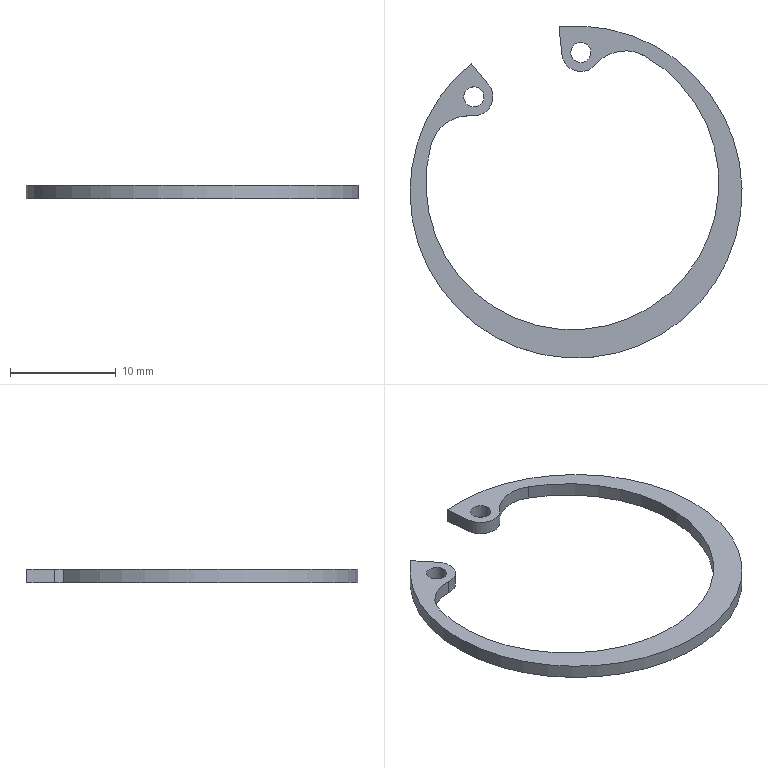Component | NX | 16 | 1 solid | 12 faces | box 31.4 x 31.4 x 1.3 mm | volume 239 mm3 | cylinder 8 | plane 4 | commonest cylinder face diameters 7.4 x2 3.6 x2 1.9 x2 27.7 x1 31.4 x1
STEP:
#1=CARTESIAN_POINT('',(0.,0.,0.));
#2=DIRECTION('',(0.,0.,1.));
#3=DIRECTION('',(1.,0.,0.));
#4=AXIS2_PLACEMENT_3D('',#1,#2,#3);
#5=CARTESIAN_POINT('',(-9.811,23.707,-49.8));
#6=VERTEX_POINT('',#5);
#7=CARTESIAN_POINT('',(-9.811,23.707,-48.5));
#8=VERTEX_POINT('',#7);
#9=CARTESIAN_POINT('',(-9.811,23.707,-49.8));
#10=DIRECTION('',(0.,0.,1.));
#11=VECTOR('',#10,1.);
#12=LINE('',#9,#11);
#13=CARTESIAN_POINT('',(-10.132,20.021,-49.8));
#14=DIRECTION('',(0.,0.,1.));
#15=DIRECTION('',(-0.9237,-0.383,0.));
#16=AXIS2_PLACEMENT_3D('',#13,#14,#15);
#17=CYLINDRICAL_SURFACE('',#16,3.7);
#18=CARTESIAN_POINT('',(4.233,0.));
#19=DIRECTION('',(0.,1.));
#20=VECTOR('',#19,1.);
#21=LINE('',#18,#20);
#22=(GEOMETRIC_REPRESENTATION_CONTEXT(2)PARAMETRIC_REPRESENTATION_CONTEXT()REPRESENTATION_CONTEXT('',''));
#23=DEFINITIONAL_REPRESENTATION('',(#21),#22);
#24=PCURVE('',#17,#23);
#25=CARTESIAN_POINT('',(-9.655,25.501,-49.8));
#26=DIRECTION('',(0.,0.,1.));
#27=DIRECTION('',(-0.9237,-0.383,0.));
#28=AXIS2_PLACEMENT_3D('',#25,#26,#27);
#29=CYLINDRICAL_SURFACE('',#28,1.8);
#30=CARTESIAN_POINT('',(1.091,0.));
#31=DIRECTION('',(0.,1.));
#32=VECTOR('',#31,1.);
#33=LINE('',#30,#32);
#34=(GEOMETRIC_REPRESENTATION_CONTEXT(2)PARAMETRIC_REPRESENTATION_CONTEXT()REPRESENTATION_CONTEXT('',''));
#35=DEFINITIONAL_REPRESENTATION('',(#33),#34);
#36=PCURVE('',#29,#35);
#37=SURFACE_CURVE('',#12,(#24,#36),.PCURVE_S1.);
#38=EDGE_CURVE('',#6,#8,#37,.T.);
#39=ORIENTED_EDGE('',*,*,#38,.F.);
#40=CARTESIAN_POINT('',(-13.699,21.002,-49.8));
#41=VERTEX_POINT('',#40);
#42=CARTESIAN_POINT('',(-10.132,20.021,-49.8));
#43=DIRECTION('',(0.,0.,1.));
#44=DIRECTION('',(0.9237,0.383,0.));
#45=AXIS2_PLACEMENT_3D('',#42,#43,#44);
#46=CIRCLE('',#45,3.7);
#47=CARTESIAN_POINT('',(3.142,0.));
#48=DIRECTION('',(1.,0.));
#49=VECTOR('',#48,1.);
#50=LINE('',#47,#49);
#51=(GEOMETRIC_REPRESENTATION_CONTEXT(2)PARAMETRIC_REPRESENTATION_CONTEXT()REPRESENTATION_CONTEXT('',''));
#52=DEFINITIONAL_REPRESENTATION('',(#50),#51);
#53=PCURVE('',#17,#52);
#54=CARTESIAN_POINT('',(-10.132,20.021,-49.8));
#55=DIRECTION('',(0.,0.,1.));
#56=DIRECTION('',(-0.9237,-0.383,0.));
#57=AXIS2_PLACEMENT_3D('',#54,#55,#56);
#58=PLANE('',#57);
#59=CARTESIAN_POINT('',(0.,0.));
#60=DIRECTION('',(-1.,0.));
#61=AXIS2_PLACEMENT_2D('',#59,#60);
#62=CIRCLE('',#61,3.7);
#63=(GEOMETRIC_REPRESENTATION_CONTEXT(2)PARAMETRIC_REPRESENTATION_CONTEXT()REPRESENTATION_CONTEXT('',''));
#64=DEFINITIONAL_REPRESENTATION('',(#62),#63);
#65=PCURVE('',#58,#64);
#66=SURFACE_CURVE('',#46,(#53,#65),.PCURVE_S1.);
#67=EDGE_CURVE('',#6,#41,#66,.T.);
#68=ORIENTED_EDGE('',*,*,#67,.T.);
#69=CARTESIAN_POINT('',(-13.699,21.002,-48.5));
#70=VERTEX_POINT('',#69);
#71=CARTESIAN_POINT('',(-13.699,21.002,-49.8));
#72=DIRECTION('',(0.,0.,1.));
#73=VECTOR('',#72,1.);
#74=LINE('',#71,#73);
#75=CARTESIAN_POINT('',(5.622,0.));
#76=DIRECTION('',(0.,1.));
#77=VECTOR('',#76,1.);
#78=LINE('',#75,#77);
#79=(GEOMETRIC_REPRESENTATION_CONTEXT(2)PARAMETRIC_REPRESENTATION_CONTEXT()REPRESENTATION_CONTEXT('',''));
#80=DEFINITIONAL_REPRESENTATION('',(#78),#79);
#81=PCURVE('',#17,#80);
#82=CARTESIAN_POINT('',(-0.3447,17.331,-49.8));
#83=DIRECTION('',(0.,0.,1.));
#84=DIRECTION('',(-0.9237,-0.383,0.));
#85=AXIS2_PLACEMENT_3D('',#82,#83,#84);
#86=CYLINDRICAL_SURFACE('',#85,13.85);
#87=CARTESIAN_POINT('',(-0.6613,0.));
#88=DIRECTION('',(0.,1.));
#89=VECTOR('',#88,1.);
#90=LINE('',#87,#89);
#91=(GEOMETRIC_REPRESENTATION_CONTEXT(2)PARAMETRIC_REPRESENTATION_CONTEXT()REPRESENTATION_CONTEXT('',''));
#92=DEFINITIONAL_REPRESENTATION('',(#90),#91);
#93=PCURVE('',#86,#92);
#94=SURFACE_CURVE('',#74,(#81,#93),.PCURVE_S1.);
#95=EDGE_CURVE('',#41,#70,#94,.T.);
#96=ORIENTED_EDGE('',*,*,#95,.T.);
#97=CARTESIAN_POINT('',(-10.132,20.021,-48.5));
#98=DIRECTION('',(0.,0.,1.));
#99=DIRECTION('',(0.9237,0.383,0.));
#100=AXIS2_PLACEMENT_3D('',#97,#98,#99);
#101=CIRCLE('',#100,3.7);
#102=CARTESIAN_POINT('',(3.142,1.3));
#103=DIRECTION('',(1.,0.));
#104=VECTOR('',#103,1.);
#105=LINE('',#102,#104);
#106=(GEOMETRIC_REPRESENTATION_CONTEXT(2)PARAMETRIC_REPRESENTATION_CONTEXT()REPRESENTATION_CONTEXT('',''));
#107=DEFINITIONAL_REPRESENTATION('',(#105),#106);
#108=PCURVE('',#17,#107);
#109=CARTESIAN_POINT('',(-10.132,20.021,-48.5));
#110=DIRECTION('',(0.,0.,1.));
#111=DIRECTION('',(-0.9237,-0.383,0.));
#112=AXIS2_PLACEMENT_3D('',#109,#110,#111);
#113=PLANE('',#112);
#114=CARTESIAN_POINT('',(0.,0.));
#115=DIRECTION('',(-1.,0.));
#116=AXIS2_PLACEMENT_2D('',#114,#115);
#117=CIRCLE('',#116,3.7);
#118=(GEOMETRIC_REPRESENTATION_CONTEXT(2)PARAMETRIC_REPRESENTATION_CONTEXT()REPRESENTATION_CONTEXT('',''));
#119=DEFINITIONAL_REPRESENTATION('',(#117),#118);
#120=PCURVE('',#113,#119);
#121=SURFACE_CURVE('',#101,(#108,#120),.PCURVE_S1.);
#122=EDGE_CURVE('',#8,#70,#121,.T.);
#123=ORIENTED_EDGE('',*,*,#122,.F.);
#124=EDGE_LOOP('',(#39,#68,#96,#123));
#125=FACE_BOUND('',#124,.F.);
#126=ADVANCED_FACE('',(#125),#17,.F.);
#127=ORIENTED_EDGE('',*,*,#95,.F.);
#128=CARTESIAN_POINT('',(6.493,29.375,-49.8));
#129=VERTEX_POINT('',#128);
#130=CARTESIAN_POINT('',(-0.3447,17.331,-49.8));
#131=DIRECTION('',(0.,0.,1.));
#132=DIRECTION('',(0.9237,0.383,0.));
#133=AXIS2_PLACEMENT_3D('',#130,#131,#132);
#134=CIRCLE('',#133,13.85);
#135=CARTESIAN_POINT('',(-3.142,0.));
#136=DIRECTION('',(1.,0.));
#137=VECTOR('',#136,1.);
#138=LINE('',#135,#137);
#139=(GEOMETRIC_REPRESENTATION_CONTEXT(2)PARAMETRIC_REPRESENTATION_CONTEXT()REPRESENTATION_CONTEXT('',''));
#140=DEFINITIONAL_REPRESENTATION('',(#138),#139);
#141=PCURVE('',#86,#140);
#142=CARTESIAN_POINT('',(-8.01,6.234));
#143=DIRECTION('',(-1.,0.));
#144=AXIS2_PLACEMENT_2D('',#142,#143);
#145=CIRCLE('',#144,13.85);
#146=(GEOMETRIC_REPRESENTATION_CONTEXT(2)PARAMETRIC_REPRESENTATION_CONTEXT()REPRESENTATION_CONTEXT('',''));
#147=DEFINITIONAL_REPRESENTATION('',(#145),#146);
#148=PCURVE('',#58,#147);
#149=SURFACE_CURVE('',#134,(#141,#148),.PCURVE_S1.);
#150=EDGE_CURVE('',#41,#129,#149,.T.);
#151=ORIENTED_EDGE('',*,*,#150,.T.);
#152=CARTESIAN_POINT('',(6.493,29.375,-48.5));
#153=VERTEX_POINT('',#152);
#154=CARTESIAN_POINT('',(6.493,29.375,-49.8));
#155=DIRECTION('',(0.,0.,1.));
#156=VECTOR('',#155,1.);
#157=LINE('',#154,#156);
#158=CARTESIAN_POINT('',(3.803,0.));
#159=DIRECTION('',(0.,1.));
#160=VECTOR('',#159,1.);
#161=LINE('',#158,#160);
#162=(GEOMETRIC_REPRESENTATION_CONTEXT(2)PARAMETRIC_REPRESENTATION_CONTEXT()REPRESENTATION_CONTEXT('',''));
#163=DEFINITIONAL_REPRESENTATION('',(#161),#162);
#164=PCURVE('',#86,#163);
#165=CARTESIAN_POINT('',(4.667,26.158,-49.8));
#166=DIRECTION('',(0.,0.,1.));
#167=DIRECTION('',(-0.9237,-0.383,0.));
#168=AXIS2_PLACEMENT_3D('',#165,#166,#167);
#169=CYLINDRICAL_SURFACE('',#168,3.7);
#170=CARTESIAN_POINT('',(3.803,0.));
#171=DIRECTION('',(0.,1.));
#172=VECTOR('',#171,1.);
#173=LINE('',#170,#172);
#174=(GEOMETRIC_REPRESENTATION_CONTEXT(2)PARAMETRIC_REPRESENTATION_CONTEXT()REPRESENTATION_CONTEXT('',''));
#175=DEFINITIONAL_REPRESENTATION('',(#173),#174);
#176=PCURVE('',#169,#175);
#177=SURFACE_CURVE('',#157,(#164,#176),.PCURVE_S1.);
#178=EDGE_CURVE('',#129,#153,#177,.T.);
#179=ORIENTED_EDGE('',*,*,#178,.T.);
#180=CARTESIAN_POINT('',(-0.3447,17.331,-48.5));
#181=DIRECTION('',(0.,0.,1.));
#182=DIRECTION('',(0.9237,0.383,0.));
#183=AXIS2_PLACEMENT_3D('',#180,#181,#182);
#184=CIRCLE('',#183,13.85);
#185=CARTESIAN_POINT('',(-3.142,1.3));
#186=DIRECTION('',(1.,0.));
#187=VECTOR('',#186,1.);
#188=LINE('',#185,#187);
#189=(GEOMETRIC_REPRESENTATION_CONTEXT(2)PARAMETRIC_REPRESENTATION_CONTEXT()REPRESENTATION_CONTEXT('',''));
#190=DEFINITIONAL_REPRESENTATION('',(#188),#189);
#191=PCURVE('',#86,#190);
#192=CARTESIAN_POINT('',(-8.01,6.234));
#193=DIRECTION('',(-1.,0.));
#194=AXIS2_PLACEMENT_2D('',#192,#193);
#195=CIRCLE('',#194,13.85);
#196=(GEOMETRIC_REPRESENTATION_CONTEXT(2)PARAMETRIC_REPRESENTATION_CONTEXT()REPRESENTATION_CONTEXT('',''));
#197=DEFINITIONAL_REPRESENTATION('',(#195),#196);
#198=PCURVE('',#113,#197);
#199=SURFACE_CURVE('',#184,(#191,#198),.PCURVE_S1.);
#200=EDGE_CURVE('',#70,#153,#199,.T.);
#201=ORIENTED_EDGE('',*,*,#200,.F.);
#202=EDGE_LOOP('',(#127,#151,#179,#201));
#203=FACE_BOUND('',#202,.F.);
#204=ADVANCED_FACE('',(#203),#86,.F.);
#205=ORIENTED_EDGE('',*,*,#178,.F.);
#206=CARTESIAN_POINT('',(1.832,28.536,-49.8));
#207=VERTEX_POINT('',#206);
#208=CARTESIAN_POINT('',(4.667,26.158,-49.8));
#209=DIRECTION('',(0.,0.,1.));
#210=DIRECTION('',(-0.9237,-0.383,0.));
#211=AXIS2_PLACEMENT_3D('',#208,#209,#210);
#212=CIRCLE('',#211,3.7);
#213=CARTESIAN_POINT('',(0.,0.));
#214=DIRECTION('',(1.,0.));
#215=VECTOR('',#214,1.);
#216=LINE('',#213,#215);
#217=(GEOMETRIC_REPRESENTATION_CONTEXT(2)PARAMETRIC_REPRESENTATION_CONTEXT()REPRESENTATION_CONTEXT('',''));
#218=DEFINITIONAL_REPRESENTATION('',(#216),#217);
#219=PCURVE('',#169,#218);
#220=CARTESIAN_POINT('',(-16.02,0.));
#221=DIRECTION('',(1.,-0.));
#222=AXIS2_PLACEMENT_2D('',#220,#221);
#223=CIRCLE('',#222,3.7);
#224=(GEOMETRIC_REPRESENTATION_CONTEXT(2)PARAMETRIC_REPRESENTATION_CONTEXT()REPRESENTATION_CONTEXT('',''));
#225=DEFINITIONAL_REPRESENTATION('',(#223),#224);
#226=PCURVE('',#58,#225);
#227=SURFACE_CURVE('',#212,(#219,#226),.PCURVE_S1.);
#228=EDGE_CURVE('',#129,#207,#227,.T.);
#229=ORIENTED_EDGE('',*,*,#228,.T.);
#230=CARTESIAN_POINT('',(1.832,28.536,-48.5));
#231=VERTEX_POINT('',#230);
#232=CARTESIAN_POINT('',(1.832,28.536,-49.8));
#233=DIRECTION('',(0.,0.,1.));
#234=VECTOR('',#233,1.);
#235=LINE('',#232,#234);
#236=CARTESIAN_POINT('',(5.192,0.));
#237=DIRECTION('',(0.,1.));
#238=VECTOR('',#237,1.);
#239=LINE('',#236,#238);
#240=(GEOMETRIC_REPRESENTATION_CONTEXT(2)PARAMETRIC_REPRESENTATION_CONTEXT()REPRESENTATION_CONTEXT('',''));
#241=DEFINITIONAL_REPRESENTATION('',(#239),#240);
#242=PCURVE('',#169,#241);
#243=CARTESIAN_POINT('',(0.4526,29.692,-49.8));
#244=DIRECTION('',(0.,0.,1.));
#245=DIRECTION('',(-0.9237,-0.383,0.));
#246=AXIS2_PLACEMENT_3D('',#243,#244,#245);
#247=CYLINDRICAL_SURFACE('',#246,1.8);
#248=CARTESIAN_POINT('',(2.051,0.));
#249=DIRECTION('',(0.,1.));
#250=VECTOR('',#249,1.);
#251=LINE('',#248,#250);
#252=(GEOMETRIC_REPRESENTATION_CONTEXT(2)PARAMETRIC_REPRESENTATION_CONTEXT()REPRESENTATION_CONTEXT('',''));
#253=DEFINITIONAL_REPRESENTATION('',(#251),#252);
#254=PCURVE('',#247,#253);
#255=SURFACE_CURVE('',#235,(#242,#254),.PCURVE_S1.);
#256=EDGE_CURVE('',#207,#231,#255,.T.);
#257=ORIENTED_EDGE('',*,*,#256,.T.);
#258=CARTESIAN_POINT('',(4.667,26.158,-48.5));
#259=DIRECTION('',(0.,0.,1.));
#260=DIRECTION('',(-0.9237,-0.383,0.));
#261=AXIS2_PLACEMENT_3D('',#258,#259,#260);
#262=CIRCLE('',#261,3.7);
#263=CARTESIAN_POINT('',(0.,1.3));
#264=DIRECTION('',(1.,0.));
#265=VECTOR('',#264,1.);
#266=LINE('',#263,#265);
#267=(GEOMETRIC_REPRESENTATION_CONTEXT(2)PARAMETRIC_REPRESENTATION_CONTEXT()REPRESENTATION_CONTEXT('',''));
#268=DEFINITIONAL_REPRESENTATION('',(#266),#267);
#269=PCURVE('',#169,#268);
#270=CARTESIAN_POINT('',(-16.02,0.));
#271=DIRECTION('',(1.,-0.));
#272=AXIS2_PLACEMENT_2D('',#270,#271);
#273=CIRCLE('',#272,3.7);
#274=(GEOMETRIC_REPRESENTATION_CONTEXT(2)PARAMETRIC_REPRESENTATION_CONTEXT()REPRESENTATION_CONTEXT('',''));
#275=DEFINITIONAL_REPRESENTATION('',(#273),#274);
#276=PCURVE('',#113,#275);
#277=SURFACE_CURVE('',#262,(#269,#276),.PCURVE_S1.);
#278=EDGE_CURVE('',#153,#231,#277,.T.);
#279=ORIENTED_EDGE('',*,*,#278,.F.);
#280=EDGE_LOOP('',(#205,#229,#257,#279));
#281=FACE_BOUND('',#280,.F.);
#282=ADVANCED_FACE('',(#281),#169,.F.);
#283=CARTESIAN_POINT('',(-1.338,29.508,-48.5));
#284=VERTEX_POINT('',#283);
#285=CARTESIAN_POINT('',(0.4526,29.692,-48.5));
#286=DIRECTION('',(0.,0.,-1.));
#287=DIRECTION('',(-0.9237,-0.383,0.));
#288=AXIS2_PLACEMENT_3D('',#285,#286,#287);
#289=CIRCLE('',#288,1.8);
#290=CARTESIAN_POINT('',(6.283,1.3));
#291=DIRECTION('',(-1.,0.));
#292=VECTOR('',#291,1.);
#293=LINE('',#290,#292);
#294=(GEOMETRIC_REPRESENTATION_CONTEXT(2)PARAMETRIC_REPRESENTATION_CONTEXT()REPRESENTATION_CONTEXT('',''));
#295=DEFINITIONAL_REPRESENTATION('',(#293),#294);
#296=PCURVE('',#247,#295);
#297=CARTESIAN_POINT('',(-11.682,-4.879));
#298=CARTESIAN_POINT('',(-11.682,-7.997));
#299=CARTESIAN_POINT('',(-14.382,-6.438));
#300=CARTESIAN_POINT('',(-17.082,-4.879));
#301=CARTESIAN_POINT('',(-14.382,-3.32));
#302=CARTESIAN_POINT('',(-11.682,-1.761));
#303=CARTESIAN_POINT('',(-11.682,-4.879));
#304=(BOUNDED_CURVE()B_SPLINE_CURVE(2,(#297,#298,#299,#300,#301,#302,#303),.UNSPECIFIED.,.T.,.F.)B_SPLINE_CURVE_WITH_KNOTS((1,2,2,2,2,1),(-2.094,0.,2.094,4.189,6.283,8.378),.UNSPECIFIED.)CURVE()GEOMETRIC_REPRESENTATION_ITEM()RATIONAL_B_SPLINE_CURVE((1.,0.5,1.,0.5,1.,0.5,1.))REPRESENTATION_ITEM(''));
#305=(GEOMETRIC_REPRESENTATION_CONTEXT(2)PARAMETRIC_REPRESENTATION_CONTEXT()REPRESENTATION_CONTEXT('',''));
#306=DEFINITIONAL_REPRESENTATION('',(#304),#305);
#307=PCURVE('',#113,#306);
#308=SURFACE_CURVE('',#289,(#296,#307),.PCURVE_S1.);
#309=EDGE_CURVE('',#231,#284,#308,.T.);
#310=ORIENTED_EDGE('',*,*,#309,.T.);
#311=CARTESIAN_POINT('',(-1.338,29.508,-49.8));
#312=VERTEX_POINT('',#311);
#313=CARTESIAN_POINT('',(-1.338,29.508,-49.8));
#314=DIRECTION('',(0.,0.,1.));
#315=VECTOR('',#314,1.);
#316=LINE('',#313,#315);
#317=CARTESIAN_POINT('',(-0.2906,0.));
#318=DIRECTION('',(0.,1.));
#319=VECTOR('',#318,1.);
#320=LINE('',#317,#319);
#321=(GEOMETRIC_REPRESENTATION_CONTEXT(2)PARAMETRIC_REPRESENTATION_CONTEXT()REPRESENTATION_CONTEXT('',''));
#322=DEFINITIONAL_REPRESENTATION('',(#320),#321);
#323=PCURVE('',#247,#322);
#324=CARTESIAN_POINT('',(-1.338,29.508,-49.8));
#325=DIRECTION('',(0.9948,0.1023,0.));
#326=DIRECTION('',(0.1023,-0.9948,0.));
#327=AXIS2_PLACEMENT_3D('',#324,#325,#326);
#328=PLANE('',#327);
#329=CARTESIAN_POINT('',(0.,0.));
#330=DIRECTION('',(0.,-1.));
#331=VECTOR('',#330,1.);
#332=LINE('',#329,#331);
#333=(GEOMETRIC_REPRESENTATION_CONTEXT(2)PARAMETRIC_REPRESENTATION_CONTEXT()REPRESENTATION_CONTEXT('',''));
#334=DEFINITIONAL_REPRESENTATION('',(#332),#333);
#335=PCURVE('',#328,#334);
#336=SURFACE_CURVE('',#316,(#323,#335),.PCURVE_S1.);
#337=EDGE_CURVE('',#312,#284,#336,.T.);
#338=ORIENTED_EDGE('',*,*,#337,.F.);
#339=CARTESIAN_POINT('',(0.4526,29.692,-49.8));
#340=DIRECTION('',(0.,0.,-1.));
#341=DIRECTION('',(-0.9237,-0.383,0.));
#342=AXIS2_PLACEMENT_3D('',#339,#340,#341);
#343=CIRCLE('',#342,1.8);
#344=CARTESIAN_POINT('',(6.283,0.));
#345=DIRECTION('',(-1.,0.));
#346=VECTOR('',#345,1.);
#347=LINE('',#344,#346);
#348=(GEOMETRIC_REPRESENTATION_CONTEXT(2)PARAMETRIC_REPRESENTATION_CONTEXT()REPRESENTATION_CONTEXT('',''));
#349=DEFINITIONAL_REPRESENTATION('',(#347),#348);
#350=PCURVE('',#247,#349);
#351=CARTESIAN_POINT('',(-11.682,-4.879));
#352=CARTESIAN_POINT('',(-11.682,-7.997));
#353=CARTESIAN_POINT('',(-14.382,-6.438));
#354=CARTESIAN_POINT('',(-17.082,-4.879));
#355=CARTESIAN_POINT('',(-14.382,-3.32));
#356=CARTESIAN_POINT('',(-11.682,-1.761));
#357=CARTESIAN_POINT('',(-11.682,-4.879));
#358=(BOUNDED_CURVE()B_SPLINE_CURVE(2,(#351,#352,#353,#354,#355,#356,#357),.UNSPECIFIED.,.T.,.F.)B_SPLINE_CURVE_WITH_KNOTS((1,2,2,2,2,1),(-2.094,0.,2.094,4.189,6.283,8.378),.UNSPECIFIED.)CURVE()GEOMETRIC_REPRESENTATION_ITEM()RATIONAL_B_SPLINE_CURVE((1.,0.5,1.,0.5,1.,0.5,1.))REPRESENTATION_ITEM(''));
#359=(GEOMETRIC_REPRESENTATION_CONTEXT(2)PARAMETRIC_REPRESENTATION_CONTEXT()REPRESENTATION_CONTEXT('',''));
#360=DEFINITIONAL_REPRESENTATION('',(#358),#359);
#361=PCURVE('',#58,#360);
#362=SURFACE_CURVE('',#343,(#350,#361),.PCURVE_S1.);
#363=EDGE_CURVE('',#207,#312,#362,.T.);
#364=ORIENTED_EDGE('',*,*,#363,.F.);
#365=ORIENTED_EDGE('',*,*,#256,.T.);
#366=EDGE_LOOP('',(#310,#338,#364,#365));
#367=FACE_BOUND('',#366,.T.);
#368=ADVANCED_FACE('',(#367),#247,.T.);
#369=CARTESIAN_POINT('',(-1.606,32.118,-48.5));
#370=VERTEX_POINT('',#369);
#371=CARTESIAN_POINT('',(-1.338,29.508,-48.5));
#372=DIRECTION('',(-0.1023,0.9948,0.));
#373=VECTOR('',#372,1.);
#374=LINE('',#371,#373);
#375=CARTESIAN_POINT('',(0.,-1.3));
#376=DIRECTION('',(-1.,0.));
#377=VECTOR('',#376,1.);
#378=LINE('',#375,#377);
#379=(GEOMETRIC_REPRESENTATION_CONTEXT(2)PARAMETRIC_REPRESENTATION_CONTEXT()REPRESENTATION_CONTEXT('',''));
#380=DEFINITIONAL_REPRESENTATION('',(#378),#379);
#381=PCURVE('',#328,#380);
#382=CARTESIAN_POINT('',(-11.757,-5.395));
#383=DIRECTION('',(-0.2865,-0.9581));
#384=VECTOR('',#383,1.);
#385=LINE('',#382,#384);
#386=(GEOMETRIC_REPRESENTATION_CONTEXT(2)PARAMETRIC_REPRESENTATION_CONTEXT()REPRESENTATION_CONTEXT('',''));
#387=DEFINITIONAL_REPRESENTATION('',(#385),#386);
#388=PCURVE('',#113,#387);
#389=SURFACE_CURVE('',#374,(#381,#388),.PCURVE_S1.);
#390=EDGE_CURVE('',#284,#370,#389,.T.);
#391=ORIENTED_EDGE('',*,*,#390,.T.);
#392=CARTESIAN_POINT('',(-1.606,32.118,-49.8));
#393=VERTEX_POINT('',#392);
#394=CARTESIAN_POINT('',(-1.606,32.118,-49.8));
#395=DIRECTION('',(0.,0.,1.));
#396=VECTOR('',#395,1.);
#397=LINE('',#394,#396);
#398=CARTESIAN_POINT('',(-2.623,0.));
#399=DIRECTION('',(0.,-1.));
#400=VECTOR('',#399,1.);
#401=LINE('',#398,#400);
#402=(GEOMETRIC_REPRESENTATION_CONTEXT(2)PARAMETRIC_REPRESENTATION_CONTEXT()REPRESENTATION_CONTEXT('',''));
#403=DEFINITIONAL_REPRESENTATION('',(#401),#402);
#404=PCURVE('',#328,#403);
#405=CARTESIAN_POINT('',(0.,16.5,-49.8));
#406=DIRECTION('',(0.,0.,1.));
#407=DIRECTION('',(-0.9237,-0.383,0.));
#408=AXIS2_PLACEMENT_3D('',#405,#406,#407);
#409=CYLINDRICAL_SURFACE('',#408,15.7);
#410=CARTESIAN_POINT('',(4.422,0.));
#411=DIRECTION('',(0.,1.));
#412=VECTOR('',#411,1.);
#413=LINE('',#410,#412);
#414=(GEOMETRIC_REPRESENTATION_CONTEXT(2)PARAMETRIC_REPRESENTATION_CONTEXT()REPRESENTATION_CONTEXT('',''));
#415=DEFINITIONAL_REPRESENTATION('',(#413),#414);
#416=PCURVE('',#409,#415);
#417=SURFACE_CURVE('',#397,(#404,#416),.PCURVE_S1.);
#418=EDGE_CURVE('',#393,#370,#417,.T.);
#419=ORIENTED_EDGE('',*,*,#418,.F.);
#420=CARTESIAN_POINT('',(-1.338,29.508,-49.8));
#421=DIRECTION('',(-0.1023,0.9948,0.));
#422=VECTOR('',#421,1.);
#423=LINE('',#420,#422);
#424=CARTESIAN_POINT('',(0.,0.));
#425=DIRECTION('',(-1.,0.));
#426=VECTOR('',#425,1.);
#427=LINE('',#424,#426);
#428=(GEOMETRIC_REPRESENTATION_CONTEXT(2)PARAMETRIC_REPRESENTATION_CONTEXT()REPRESENTATION_CONTEXT('',''));
#429=DEFINITIONAL_REPRESENTATION('',(#427),#428);
#430=PCURVE('',#328,#429);
#431=CARTESIAN_POINT('',(-11.757,-5.395));
#432=DIRECTION('',(-0.2865,-0.9581));
#433=VECTOR('',#432,1.);
#434=LINE('',#431,#433);
#435=(GEOMETRIC_REPRESENTATION_CONTEXT(2)PARAMETRIC_REPRESENTATION_CONTEXT()REPRESENTATION_CONTEXT('',''));
#436=DEFINITIONAL_REPRESENTATION('',(#434),#435);
#437=PCURVE('',#58,#436);
#438=SURFACE_CURVE('',#423,(#430,#437),.PCURVE_S1.);
#439=EDGE_CURVE('',#312,#393,#438,.T.);
#440=ORIENTED_EDGE('',*,*,#439,.F.);
#441=ORIENTED_EDGE('',*,*,#337,.T.);
#442=EDGE_LOOP('',(#391,#419,#440,#441));
#443=FACE_BOUND('',#442,.T.);
#444=ADVANCED_FACE('',(#443),#328,.F.);
#445=CARTESIAN_POINT('',(-9.917,28.671,-48.5));
#446=VERTEX_POINT('',#445);
#447=CARTESIAN_POINT('',(0.,16.5,-48.5));
#448=DIRECTION('',(0.,0.,-1.));
#449=DIRECTION('',(0.9237,0.383,0.));
#450=AXIS2_PLACEMENT_3D('',#447,#448,#449);
#451=CIRCLE('',#450,15.7);
#452=CARTESIAN_POINT('',(9.425,1.3));
#453=DIRECTION('',(-1.,0.));
#454=VECTOR('',#453,1.);
#455=LINE('',#452,#454);
#456=(GEOMETRIC_REPRESENTATION_CONTEXT(2)PARAMETRIC_REPRESENTATION_CONTEXT()REPRESENTATION_CONTEXT('',''));
#457=DEFINITIONAL_REPRESENTATION('',(#455),#456);
#458=PCURVE('',#409,#457);
#459=CARTESIAN_POINT('',(-23.71,7.134));
#460=CARTESIAN_POINT('',(-23.71,34.327));
#461=CARTESIAN_POINT('',(-0.1602,20.73));
#462=CARTESIAN_POINT('',(23.39,7.134));
#463=CARTESIAN_POINT('',(-0.1602,-6.463));
#464=CARTESIAN_POINT('',(-23.71,-20.059));
#465=CARTESIAN_POINT('',(-23.71,7.134));
#466=(BOUNDED_CURVE()B_SPLINE_CURVE(2,(#459,#460,#461,#462,#463,#464,#465),.UNSPECIFIED.,.T.,.F.)B_SPLINE_CURVE_WITH_KNOTS((1,2,2,2,2,1),(-2.094,0.,2.094,4.189,6.283,8.378),.UNSPECIFIED.)CURVE()GEOMETRIC_REPRESENTATION_ITEM()RATIONAL_B_SPLINE_CURVE((1.,0.5,1.,0.5,1.,0.5,1.))REPRESENTATION_ITEM(''));
#467=(GEOMETRIC_REPRESENTATION_CONTEXT(2)PARAMETRIC_REPRESENTATION_CONTEXT()REPRESENTATION_CONTEXT('',''));
#468=DEFINITIONAL_REPRESENTATION('',(#466),#467);
#469=PCURVE('',#113,#468);
#470=SURFACE_CURVE('',#451,(#458,#469),.PCURVE_S1.);
#471=EDGE_CURVE('',#370,#446,#470,.T.);
#472=ORIENTED_EDGE('',*,*,#471,.T.);
#473=CARTESIAN_POINT('',(-9.917,28.671,-49.8));
#474=VERTEX_POINT('',#473);
#475=CARTESIAN_POINT('',(-9.917,28.671,-49.8));
#476=DIRECTION('',(0.,0.,1.));
#477=VECTOR('',#476,1.);
#478=LINE('',#475,#477);
#479=CARTESIAN_POINT('',(-1.28,0.));
#480=DIRECTION('',(0.,1.));
#481=VECTOR('',#480,1.);
#482=LINE('',#479,#481);
#483=(GEOMETRIC_REPRESENTATION_CONTEXT(2)PARAMETRIC_REPRESENTATION_CONTEXT()REPRESENTATION_CONTEXT('',''));
#484=DEFINITIONAL_REPRESENTATION('',(#482),#483);
#485=PCURVE('',#409,#484);
#486=CARTESIAN_POINT('',(-9.917,28.671,-49.8));
#487=DIRECTION('',(-0.7752,-0.6317,0.));
#488=DIRECTION('',(-0.6317,0.7752,0.));
#489=AXIS2_PLACEMENT_3D('',#486,#487,#488);
#490=PLANE('',#489);
#491=CARTESIAN_POINT('',(0.,0.));
#492=DIRECTION('',(0.,-1.));
#493=VECTOR('',#492,1.);
#494=LINE('',#491,#493);
#495=(GEOMETRIC_REPRESENTATION_CONTEXT(2)PARAMETRIC_REPRESENTATION_CONTEXT()REPRESENTATION_CONTEXT('',''));
#496=DEFINITIONAL_REPRESENTATION('',(#494),#495);
#497=PCURVE('',#490,#496);
#498=SURFACE_CURVE('',#478,(#485,#497),.PCURVE_S1.);
#499=EDGE_CURVE('',#474,#446,#498,.T.);
#500=ORIENTED_EDGE('',*,*,#499,.F.);
#501=CARTESIAN_POINT('',(0.,16.5,-49.8));
#502=DIRECTION('',(0.,0.,-1.));
#503=DIRECTION('',(0.9237,0.383,0.));
#504=AXIS2_PLACEMENT_3D('',#501,#502,#503);
#505=CIRCLE('',#504,15.7);
#506=CARTESIAN_POINT('',(9.425,0.));
#507=DIRECTION('',(-1.,0.));
#508=VECTOR('',#507,1.);
#509=LINE('',#506,#508);
#510=(GEOMETRIC_REPRESENTATION_CONTEXT(2)PARAMETRIC_REPRESENTATION_CONTEXT()REPRESENTATION_CONTEXT('',''));
#511=DEFINITIONAL_REPRESENTATION('',(#509),#510);
#512=PCURVE('',#409,#511);
#513=CARTESIAN_POINT('',(-23.71,7.134));
#514=CARTESIAN_POINT('',(-23.71,34.327));
#515=CARTESIAN_POINT('',(-0.1602,20.73));
#516=CARTESIAN_POINT('',(23.39,7.134));
#517=CARTESIAN_POINT('',(-0.1602,-6.463));
#518=CARTESIAN_POINT('',(-23.71,-20.059));
#519=CARTESIAN_POINT('',(-23.71,7.134));
#520=(BOUNDED_CURVE()B_SPLINE_CURVE(2,(#513,#514,#515,#516,#517,#518,#519),.UNSPECIFIED.,.T.,.F.)B_SPLINE_CURVE_WITH_KNOTS((1,2,2,2,2,1),(-2.094,0.,2.094,4.189,6.283,8.378),.UNSPECIFIED.)CURVE()GEOMETRIC_REPRESENTATION_ITEM()RATIONAL_B_SPLINE_CURVE((1.,0.5,1.,0.5,1.,0.5,1.))REPRESENTATION_ITEM(''));
#521=(GEOMETRIC_REPRESENTATION_CONTEXT(2)PARAMETRIC_REPRESENTATION_CONTEXT()REPRESENTATION_CONTEXT('',''));
#522=DEFINITIONAL_REPRESENTATION('',(#520),#521);
#523=PCURVE('',#58,#522);
#524=SURFACE_CURVE('',#505,(#512,#523),.PCURVE_S1.);
#525=EDGE_CURVE('',#393,#474,#524,.T.);
#526=ORIENTED_EDGE('',*,*,#525,.F.);
#527=ORIENTED_EDGE('',*,*,#418,.T.);
#528=EDGE_LOOP('',(#472,#500,#526,#527));
#529=FACE_BOUND('',#528,.T.);
#530=ADVANCED_FACE('',(#529),#409,.T.);
#531=CARTESIAN_POINT('',(-8.26,26.638,-48.5));
#532=VERTEX_POINT('',#531);
#533=CARTESIAN_POINT('',(-9.917,28.671,-48.5));
#534=DIRECTION('',(0.6317,-0.7752,0.));
#535=VECTOR('',#534,1.);
#536=LINE('',#533,#535);
#537=CARTESIAN_POINT('',(0.,-1.3));
#538=DIRECTION('',(-1.,0.));
#539=VECTOR('',#538,1.);
#540=LINE('',#537,#539);
#541=(GEOMETRIC_REPRESENTATION_CONTEXT(2)PARAMETRIC_REPRESENTATION_CONTEXT()REPRESENTATION_CONTEXT('',''));
#542=DEFINITIONAL_REPRESENTATION('',(#540),#541);
#543=PCURVE('',#490,#542);
#544=CARTESIAN_POINT('',(-3.512,-7.908));
#545=DIRECTION('',(-0.2865,0.9581));
#546=VECTOR('',#545,1.);
#547=LINE('',#544,#546);
#548=(GEOMETRIC_REPRESENTATION_CONTEXT(2)PARAMETRIC_REPRESENTATION_CONTEXT()REPRESENTATION_CONTEXT('',''));
#549=DEFINITIONAL_REPRESENTATION('',(#547),#548);
#550=PCURVE('',#113,#549);
#551=SURFACE_CURVE('',#536,(#543,#550),.PCURVE_S1.);
#552=EDGE_CURVE('',#446,#532,#551,.T.);
#553=ORIENTED_EDGE('',*,*,#552,.T.);
#554=CARTESIAN_POINT('',(-8.26,26.638,-49.8));
#555=VERTEX_POINT('',#554);
#556=CARTESIAN_POINT('',(-8.26,26.638,-49.8));
#557=DIRECTION('',(0.,0.,1.));
#558=VECTOR('',#557,1.);
#559=LINE('',#556,#558);
#560=CARTESIAN_POINT('',(-2.623,0.));
#561=DIRECTION('',(0.,-1.));
#562=VECTOR('',#561,1.);
#563=LINE('',#560,#562);
#564=(GEOMETRIC_REPRESENTATION_CONTEXT(2)PARAMETRIC_REPRESENTATION_CONTEXT()REPRESENTATION_CONTEXT('',''));
#565=DEFINITIONAL_REPRESENTATION('',(#563),#564);
#566=PCURVE('',#490,#565);
#567=CARTESIAN_POINT('',(3.432,0.));
#568=DIRECTION('',(0.,1.));
#569=VECTOR('',#568,1.);
#570=LINE('',#567,#569);
#571=(GEOMETRIC_REPRESENTATION_CONTEXT(2)PARAMETRIC_REPRESENTATION_CONTEXT()REPRESENTATION_CONTEXT('',''));
#572=DEFINITIONAL_REPRESENTATION('',(#570),#571);
#573=PCURVE('',#29,#572);
#574=SURFACE_CURVE('',#559,(#566,#573),.PCURVE_S1.);
#575=EDGE_CURVE('',#555,#532,#574,.T.);
#576=ORIENTED_EDGE('',*,*,#575,.F.);
#577=CARTESIAN_POINT('',(-9.917,28.671,-49.8));
#578=DIRECTION('',(0.6317,-0.7752,0.));
#579=VECTOR('',#578,1.);
#580=LINE('',#577,#579);
#581=CARTESIAN_POINT('',(0.,0.));
#582=DIRECTION('',(-1.,0.));
#583=VECTOR('',#582,1.);
#584=LINE('',#581,#583);
#585=(GEOMETRIC_REPRESENTATION_CONTEXT(2)PARAMETRIC_REPRESENTATION_CONTEXT()REPRESENTATION_CONTEXT('',''));
#586=DEFINITIONAL_REPRESENTATION('',(#584),#585);
#587=PCURVE('',#490,#586);
#588=CARTESIAN_POINT('',(-3.512,-7.908));
#589=DIRECTION('',(-0.2865,0.9581));
#590=VECTOR('',#589,1.);
#591=LINE('',#588,#590);
#592=(GEOMETRIC_REPRESENTATION_CONTEXT(2)PARAMETRIC_REPRESENTATION_CONTEXT()REPRESENTATION_CONTEXT('',''));
#593=DEFINITIONAL_REPRESENTATION('',(#591),#592);
#594=PCURVE('',#58,#593);
#595=SURFACE_CURVE('',#580,(#587,#594),.PCURVE_S1.);
#596=EDGE_CURVE('',#474,#555,#595,.T.);
#597=ORIENTED_EDGE('',*,*,#596,.F.);
#598=ORIENTED_EDGE('',*,*,#499,.T.);
#599=EDGE_LOOP('',(#553,#576,#597,#598));
#600=FACE_BOUND('',#599,.T.);
#601=ADVANCED_FACE('',(#600),#490,.F.);
#602=CARTESIAN_POINT('',(-0.425,29.328,-49.8));
#603=VERTEX_POINT('',#602);
#604=CARTESIAN_POINT('',(0.4526,29.692,-49.8));
#605=DIRECTION('',(0.,0.,1.));
#606=DIRECTION('',(-0.9237,-0.383,0.));
#607=AXIS2_PLACEMENT_3D('',#604,#605,#606);
#608=CIRCLE('',#607,0.95);
#609=CARTESIAN_POINT('',(0.4526,29.692,-49.8));
#610=DIRECTION('',(0.,0.,1.));
#611=DIRECTION('',(-0.9237,-0.383,0.));
#612=AXIS2_PLACEMENT_3D('',#609,#610,#611);
#613=CYLINDRICAL_SURFACE('',#612,0.95);
#614=CARTESIAN_POINT('',(0.,0.));
#615=DIRECTION('',(1.,0.));
#616=VECTOR('',#615,1.);
#617=LINE('',#614,#616);
#618=(GEOMETRIC_REPRESENTATION_CONTEXT(2)PARAMETRIC_REPRESENTATION_CONTEXT()REPRESENTATION_CONTEXT('',''));
#619=DEFINITIONAL_REPRESENTATION('',(#617),#618);
#620=PCURVE('',#613,#619);
#621=CARTESIAN_POINT('',(-13.482,-4.879));
#622=DIRECTION('',(1.,0.));
#623=AXIS2_PLACEMENT_2D('',#621,#622);
#624=CIRCLE('',#623,0.95);
#625=(GEOMETRIC_REPRESENTATION_CONTEXT(2)PARAMETRIC_REPRESENTATION_CONTEXT()REPRESENTATION_CONTEXT('',''));
#626=DEFINITIONAL_REPRESENTATION('',(#624),#625);
#627=PCURVE('',#58,#626);
#628=SURFACE_CURVE('',#608,(#620,#627),.PCURVE_S1.);
#629=EDGE_CURVE('',#603,#603,#628,.T.);
#630=ORIENTED_EDGE('',*,*,#629,.T.);
#631=CARTESIAN_POINT('',(-0.425,29.328,-48.5));
#632=VERTEX_POINT('',#631);
#633=CARTESIAN_POINT('',(-0.425,29.328,-49.8));
#634=CARTESIAN_POINT('',(-0.425,29.328,-48.5));
#635=B_SPLINE_CURVE_WITH_KNOTS('',1,(#633,#634),.UNSPECIFIED.,.F.,.F.,(2,2),(0.,1.3),.PIECEWISE_BEZIER_KNOTS.);
#636=CARTESIAN_POINT('',(6.283,0.));
#637=DIRECTION('',(0.,1.));
#638=VECTOR('',#637,1.);
#639=LINE('',#636,#638);
#640=(GEOMETRIC_REPRESENTATION_CONTEXT(2)PARAMETRIC_REPRESENTATION_CONTEXT()REPRESENTATION_CONTEXT('',''));
#641=DEFINITIONAL_REPRESENTATION('',(#639),#640);
#642=PCURVE('',#613,#641);
#643=CARTESIAN_POINT('',(0.,0.));
#644=DIRECTION('',(0.,1.));
#645=VECTOR('',#644,1.);
#646=LINE('',#643,#645);
#647=(GEOMETRIC_REPRESENTATION_CONTEXT(2)PARAMETRIC_REPRESENTATION_CONTEXT()REPRESENTATION_CONTEXT('',''));
#648=DEFINITIONAL_REPRESENTATION('',(#646),#647);
#649=PCURVE('',#613,#648);
#650=SEAM_CURVE('',#635,(#642,#649),.PCURVE_S1.);
#651=EDGE_CURVE('',#603,#632,#650,.T.);
#652=ORIENTED_EDGE('',*,*,#651,.T.);
#653=CARTESIAN_POINT('',(0.4526,29.692,-48.5));
#654=DIRECTION('',(0.,0.,1.));
#655=DIRECTION('',(-0.9237,-0.383,0.));
#656=AXIS2_PLACEMENT_3D('',#653,#654,#655);
#657=CIRCLE('',#656,0.95);
#658=CARTESIAN_POINT('',(0.,1.3));
#659=DIRECTION('',(1.,0.));
#660=VECTOR('',#659,1.);
#661=LINE('',#658,#660);
#662=(GEOMETRIC_REPRESENTATION_CONTEXT(2)PARAMETRIC_REPRESENTATION_CONTEXT()REPRESENTATION_CONTEXT('',''));
#663=DEFINITIONAL_REPRESENTATION('',(#661),#662);
#664=PCURVE('',#613,#663);
#665=CARTESIAN_POINT('',(-13.482,-4.879));
#666=DIRECTION('',(1.,0.));
#667=AXIS2_PLACEMENT_2D('',#665,#666);
#668=CIRCLE('',#667,0.95);
#669=(GEOMETRIC_REPRESENTATION_CONTEXT(2)PARAMETRIC_REPRESENTATION_CONTEXT()REPRESENTATION_CONTEXT('',''));
#670=DEFINITIONAL_REPRESENTATION('',(#668),#669);
#671=PCURVE('',#113,#670);
#672=SURFACE_CURVE('',#657,(#664,#671),.PCURVE_S1.);
#673=EDGE_CURVE('',#632,#632,#672,.T.);
#674=ORIENTED_EDGE('',*,*,#673,.F.);
#675=ORIENTED_EDGE('',*,*,#651,.F.);
#676=EDGE_LOOP('',(#630,#652,#674,#675));
#677=FACE_BOUND('',#676,.F.);
#678=ADVANCED_FACE('',(#677),#613,.F.);
#679=CARTESIAN_POINT('',(-9.655,25.501,-48.5));
#680=DIRECTION('',(0.,0.,-1.));
#681=DIRECTION('',(0.9237,0.383,0.));
#682=AXIS2_PLACEMENT_3D('',#679,#680,#681);
#683=CIRCLE('',#682,1.8);
#684=CARTESIAN_POINT('',(9.425,1.3));
#685=DIRECTION('',(-1.,0.));
#686=VECTOR('',#685,1.);
#687=LINE('',#684,#686);
#688=(GEOMETRIC_REPRESENTATION_CONTEXT(2)PARAMETRIC_REPRESENTATION_CONTEXT()REPRESENTATION_CONTEXT('',''));
#689=DEFINITIONAL_REPRESENTATION('',(#687),#688);
#690=PCURVE('',#29,#689);
#691=CARTESIAN_POINT('',(-4.339,-4.879));
#692=CARTESIAN_POINT('',(-4.339,-1.761));
#693=CARTESIAN_POINT('',(-1.639,-3.32));
#694=CARTESIAN_POINT('',(1.061,-4.879));
#695=CARTESIAN_POINT('',(-1.639,-6.438));
#696=CARTESIAN_POINT('',(-4.339,-7.997));
#697=CARTESIAN_POINT('',(-4.339,-4.879));
#698=(BOUNDED_CURVE()B_SPLINE_CURVE(2,(#691,#692,#693,#694,#695,#696,#697),.UNSPECIFIED.,.T.,.F.)B_SPLINE_CURVE_WITH_KNOTS((1,2,2,2,2,1),(-2.094,0.,2.094,4.189,6.283,8.378),.UNSPECIFIED.)CURVE()GEOMETRIC_REPRESENTATION_ITEM()RATIONAL_B_SPLINE_CURVE((1.,0.5,1.,0.5,1.,0.5,1.))REPRESENTATION_ITEM(''));
#699=(GEOMETRIC_REPRESENTATION_CONTEXT(2)PARAMETRIC_REPRESENTATION_CONTEXT()REPRESENTATION_CONTEXT('',''));
#700=DEFINITIONAL_REPRESENTATION('',(#698),#699);
#701=PCURVE('',#113,#700);
#702=SURFACE_CURVE('',#683,(#690,#701),.PCURVE_S1.);
#703=EDGE_CURVE('',#532,#8,#702,.T.);
#704=ORIENTED_EDGE('',*,*,#703,.T.);
#705=ORIENTED_EDGE('',*,*,#38,.F.);
#706=CARTESIAN_POINT('',(-9.655,25.501,-49.8));
#707=DIRECTION('',(0.,0.,-1.));
#708=DIRECTION('',(0.9237,0.383,0.));
#709=AXIS2_PLACEMENT_3D('',#706,#707,#708);
#710=CIRCLE('',#709,1.8);
#711=CARTESIAN_POINT('',(9.425,0.));
#712=DIRECTION('',(-1.,0.));
#713=VECTOR('',#712,1.);
#714=LINE('',#711,#713);
#715=(GEOMETRIC_REPRESENTATION_CONTEXT(2)PARAMETRIC_REPRESENTATION_CONTEXT()REPRESENTATION_CONTEXT('',''));
#716=DEFINITIONAL_REPRESENTATION('',(#714),#715);
#717=PCURVE('',#29,#716);
#718=CARTESIAN_POINT('',(-4.339,-4.879));
#719=CARTESIAN_POINT('',(-4.339,-1.761));
#720=CARTESIAN_POINT('',(-1.639,-3.32));
#721=CARTESIAN_POINT('',(1.061,-4.879));
#722=CARTESIAN_POINT('',(-1.639,-6.438));
#723=CARTESIAN_POINT('',(-4.339,-7.997));
#724=CARTESIAN_POINT('',(-4.339,-4.879));
#725=(BOUNDED_CURVE()B_SPLINE_CURVE(2,(#718,#719,#720,#721,#722,#723,#724),.UNSPECIFIED.,.T.,.F.)B_SPLINE_CURVE_WITH_KNOTS((1,2,2,2,2,1),(-2.094,0.,2.094,4.189,6.283,8.378),.UNSPECIFIED.)CURVE()GEOMETRIC_REPRESENTATION_ITEM()RATIONAL_B_SPLINE_CURVE((1.,0.5,1.,0.5,1.,0.5,1.))REPRESENTATION_ITEM(''));
#726=(GEOMETRIC_REPRESENTATION_CONTEXT(2)PARAMETRIC_REPRESENTATION_CONTEXT()REPRESENTATION_CONTEXT('',''));
#727=DEFINITIONAL_REPRESENTATION('',(#725),#726);
#728=PCURVE('',#58,#727);
#729=SURFACE_CURVE('',#710,(#717,#728),.PCURVE_S1.);
#730=EDGE_CURVE('',#555,#6,#729,.T.);
#731=ORIENTED_EDGE('',*,*,#730,.F.);
#732=ORIENTED_EDGE('',*,*,#575,.T.);
#733=EDGE_LOOP('',(#704,#705,#731,#732));
#734=FACE_BOUND('',#733,.T.);
#735=ADVANCED_FACE('',(#734),#29,.T.);
#736=CARTESIAN_POINT('',(-8.778,25.865,-49.8));
#737=VERTEX_POINT('',#736);
#738=CARTESIAN_POINT('',(-9.655,25.501,-49.8));
#739=DIRECTION('',(0.,0.,-1.));
#740=DIRECTION('',(0.9237,0.383,0.));
#741=AXIS2_PLACEMENT_3D('',#738,#739,#740);
#742=CIRCLE('',#741,0.95);
#743=CARTESIAN_POINT('',(-9.655,25.501,-49.8));
#744=DIRECTION('',(0.,0.,1.));
#745=DIRECTION('',(-0.9237,-0.383,0.));
#746=AXIS2_PLACEMENT_3D('',#743,#744,#745);
#747=CYLINDRICAL_SURFACE('',#746,0.95);
#748=CARTESIAN_POINT('',(9.425,0.));
#749=DIRECTION('',(-1.,0.));
#750=VECTOR('',#749,1.);
#751=LINE('',#748,#750);
#752=(GEOMETRIC_REPRESENTATION_CONTEXT(2)PARAMETRIC_REPRESENTATION_CONTEXT()REPRESENTATION_CONTEXT('',''));
#753=DEFINITIONAL_REPRESENTATION('',(#751),#752);
#754=PCURVE('',#747,#753);
#755=CARTESIAN_POINT('',(-3.489,-4.879));
#756=CARTESIAN_POINT('',(-3.489,-3.234));
#757=CARTESIAN_POINT('',(-2.064,-4.056));
#758=CARTESIAN_POINT('',(-0.6389,-4.879));
#759=CARTESIAN_POINT('',(-2.064,-5.702));
#760=CARTESIAN_POINT('',(-3.489,-6.524));
#761=CARTESIAN_POINT('',(-3.489,-4.879));
#762=(BOUNDED_CURVE()B_SPLINE_CURVE(2,(#755,#756,#757,#758,#759,#760,#761),.UNSPECIFIED.,.T.,.F.)B_SPLINE_CURVE_WITH_KNOTS((1,2,2,2,2,1),(-2.094,0.,2.094,4.189,6.283,8.378),.UNSPECIFIED.)CURVE()GEOMETRIC_REPRESENTATION_ITEM()RATIONAL_B_SPLINE_CURVE((1.,0.5,1.,0.5,1.,0.5,1.))REPRESENTATION_ITEM(''));
#763=(GEOMETRIC_REPRESENTATION_CONTEXT(2)PARAMETRIC_REPRESENTATION_CONTEXT()REPRESENTATION_CONTEXT('',''));
#764=DEFINITIONAL_REPRESENTATION('',(#762),#763);
#765=PCURVE('',#58,#764);
#766=SURFACE_CURVE('',#742,(#754,#765),.PCURVE_S1.);
#767=EDGE_CURVE('',#737,#737,#766,.T.);
#768=ORIENTED_EDGE('',*,*,#767,.F.);
#769=CARTESIAN_POINT('',(-8.778,25.865,-48.5));
#770=VERTEX_POINT('',#769);
#771=CARTESIAN_POINT('',(-8.778,25.865,-49.8));
#772=CARTESIAN_POINT('',(-8.778,25.865,-48.5));
#773=B_SPLINE_CURVE_WITH_KNOTS('',1,(#771,#772),.UNSPECIFIED.,.F.,.F.,(2,2),(0.,1.3),.PIECEWISE_BEZIER_KNOTS.);
#774=CARTESIAN_POINT('',(9.425,0.));
#775=DIRECTION('',(0.,1.));
#776=VECTOR('',#775,1.);
#777=LINE('',#774,#776);
#778=(GEOMETRIC_REPRESENTATION_CONTEXT(2)PARAMETRIC_REPRESENTATION_CONTEXT()REPRESENTATION_CONTEXT('',''));
#779=DEFINITIONAL_REPRESENTATION('',(#777),#778);
#780=PCURVE('',#747,#779);
#781=CARTESIAN_POINT('',(3.142,0.));
#782=DIRECTION('',(0.,1.));
#783=VECTOR('',#782,1.);
#784=LINE('',#781,#783);
#785=(GEOMETRIC_REPRESENTATION_CONTEXT(2)PARAMETRIC_REPRESENTATION_CONTEXT()REPRESENTATION_CONTEXT('',''));
#786=DEFINITIONAL_REPRESENTATION('',(#784),#785);
#787=PCURVE('',#747,#786);
#788=SEAM_CURVE('',#773,(#780,#787),.PCURVE_S1.);
#789=EDGE_CURVE('',#737,#770,#788,.T.);
#790=ORIENTED_EDGE('',*,*,#789,.T.);
#791=CARTESIAN_POINT('',(-9.655,25.501,-48.5));
#792=DIRECTION('',(0.,0.,-1.));
#793=DIRECTION('',(0.9237,0.383,0.));
#794=AXIS2_PLACEMENT_3D('',#791,#792,#793);
#795=CIRCLE('',#794,0.95);
#796=CARTESIAN_POINT('',(9.425,1.3));
#797=DIRECTION('',(-1.,0.));
#798=VECTOR('',#797,1.);
#799=LINE('',#796,#798);
#800=(GEOMETRIC_REPRESENTATION_CONTEXT(2)PARAMETRIC_REPRESENTATION_CONTEXT()REPRESENTATION_CONTEXT('',''));
#801=DEFINITIONAL_REPRESENTATION('',(#799),#800);
#802=PCURVE('',#747,#801);
#803=CARTESIAN_POINT('',(-3.489,-4.879));
#804=CARTESIAN_POINT('',(-3.489,-3.234));
#805=CARTESIAN_POINT('',(-2.064,-4.056));
#806=CARTESIAN_POINT('',(-0.6389,-4.879));
#807=CARTESIAN_POINT('',(-2.064,-5.702));
#808=CARTESIAN_POINT('',(-3.489,-6.524));
#809=CARTESIAN_POINT('',(-3.489,-4.879));
#810=(BOUNDED_CURVE()B_SPLINE_CURVE(2,(#803,#804,#805,#806,#807,#808,#809),.UNSPECIFIED.,.T.,.F.)B_SPLINE_CURVE_WITH_KNOTS((1,2,2,2,2,1),(-2.094,0.,2.094,4.189,6.283,8.378),.UNSPECIFIED.)CURVE()GEOMETRIC_REPRESENTATION_ITEM()RATIONAL_B_SPLINE_CURVE((1.,0.5,1.,0.5,1.,0.5,1.))REPRESENTATION_ITEM(''));
#811=(GEOMETRIC_REPRESENTATION_CONTEXT(2)PARAMETRIC_REPRESENTATION_CONTEXT()REPRESENTATION_CONTEXT('',''));
#812=DEFINITIONAL_REPRESENTATION('',(#810),#811);
#813=PCURVE('',#113,#812);
#814=SURFACE_CURVE('',#795,(#802,#813),.PCURVE_S1.);
#815=EDGE_CURVE('',#770,#770,#814,.T.);
#816=ORIENTED_EDGE('',*,*,#815,.T.);
#817=ORIENTED_EDGE('',*,*,#789,.F.);
#818=EDGE_LOOP('',(#768,#790,#816,#817));
#819=FACE_BOUND('',#818,.F.);
#820=ADVANCED_FACE('',(#819),#747,.F.);
#821=ORIENTED_EDGE('',*,*,#67,.T.);
#822=ORIENTED_EDGE('',*,*,#150,.T.);
#823=ORIENTED_EDGE('',*,*,#228,.T.);
#824=ORIENTED_EDGE('',*,*,#363,.T.);
#825=ORIENTED_EDGE('',*,*,#439,.T.);
#826=ORIENTED_EDGE('',*,*,#525,.T.);
#827=ORIENTED_EDGE('',*,*,#596,.T.);
#828=ORIENTED_EDGE('',*,*,#730,.T.);
#829=EDGE_LOOP('',(#821,#822,#823,#824,#825,#826,#827,#828));
#830=FACE_BOUND('',#829,.T.);
#831=ORIENTED_EDGE('',*,*,#629,.T.);
#832=EDGE_LOOP('',(#831));
#833=FACE_BOUND('',#832,.T.);
#834=ORIENTED_EDGE('',*,*,#767,.F.);
#835=EDGE_LOOP('',(#834));
#836=FACE_BOUND('',#835,.T.);
#837=ADVANCED_FACE('',(#830,#833,#836),#58,.F.);
#838=ORIENTED_EDGE('',*,*,#122,.F.);
#839=ORIENTED_EDGE('',*,*,#703,.F.);
#840=ORIENTED_EDGE('',*,*,#552,.F.);
#841=ORIENTED_EDGE('',*,*,#471,.F.);
#842=ORIENTED_EDGE('',*,*,#390,.F.);
#843=ORIENTED_EDGE('',*,*,#309,.F.);
#844=ORIENTED_EDGE('',*,*,#278,.F.);
#845=ORIENTED_EDGE('',*,*,#200,.F.);
#846=EDGE_LOOP('',(#838,#839,#840,#841,#842,#843,#844,#845));
#847=FACE_BOUND('',#846,.T.);
#848=ORIENTED_EDGE('',*,*,#673,.F.);
#849=EDGE_LOOP('',(#848));
#850=FACE_BOUND('',#849,.T.);
#851=ORIENTED_EDGE('',*,*,#815,.T.);
#852=EDGE_LOOP('',(#851));
#853=FACE_BOUND('',#852,.T.);
#854=ADVANCED_FACE('',(#847,#850,#853),#113,.T.);
#855=CLOSED_SHELL('',(#126,#204,#282,#368,#444,#530,#601,#678,#735,#820,#837,#854));
#856=MANIFOLD_SOLID_BREP('',#855);
#857=(LENGTH_UNIT()NAMED_UNIT(*)SI_UNIT(.MILLI.,.METRE.));
#858=UNCERTAINTY_MEASURE_WITH_UNIT(LENGTH_MEASURE(0.000002),#857,'','');
#859=(NAMED_UNIT(*)PLANE_ANGLE_UNIT()SI_UNIT($,.RADIAN.));
#860=(NAMED_UNIT(*)SI_UNIT($,.STERADIAN.)SOLID_ANGLE_UNIT());
#861=(GEOMETRIC_REPRESENTATION_CONTEXT(3)GLOBAL_UNCERTAINTY_ASSIGNED_CONTEXT((#858))GLOBAL_UNIT_ASSIGNED_CONTEXT((#857,#859,#860))REPRESENTATION_CONTEXT('',''));
#862=ADVANCED_BREP_SHAPE_REPRESENTATION('',(#4,#856),#861);